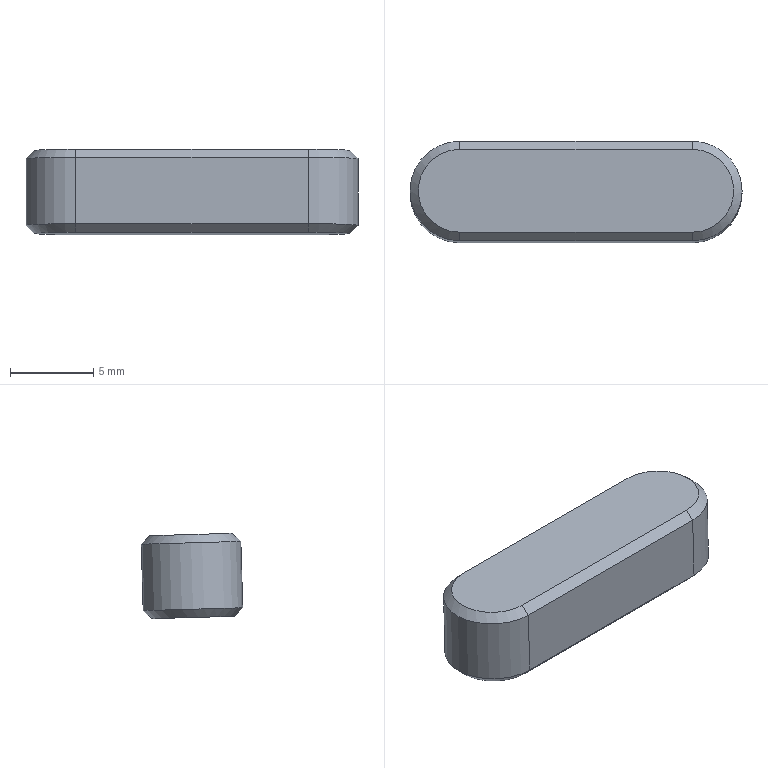Component | NX | KEY | 1 solid | 14 faces | box 20 x 6.11 x 5.14 mm | volume 550 mm3 | plane 8 | cone 4 | cylinder 2 | commonest cylinder face diameters 6 x2
STEP:
#1=CARTESIAN_POINT('',(0.,0.,0.));
#2=DIRECTION('',(0.,0.,1.));
#3=DIRECTION('',(1.,0.,0.));
#4=AXIS2_PLACEMENT_3D('',#1,#2,#3);
#5=CARTESIAN_POINT('',(-86.,-3.299,-0.9099));
#6=VERTEX_POINT('',#5);
#7=CARTESIAN_POINT('',(-86.,-3.185,3.088));
#8=VERTEX_POINT('',#7);
#9=CARTESIAN_POINT('',(-86.,-3.313,-1.41));
#10=DIRECTION('',(0.,0.0286,0.9996));
#11=VECTOR('',#10,1.);
#12=LINE('',#9,#11);
#13=CARTESIAN_POINT('',(-100.,-3.313,-1.41));
#14=DIRECTION('',(-0.,-0.9996,0.0286));
#15=DIRECTION('',(-1.,0.,-0.));
#16=AXIS2_PLACEMENT_3D('',#13,#14,#15);
#17=PLANE('',#16);
#18=CARTESIAN_POINT('',(-14.,0.));
#19=DIRECTION('',(0.,-1.));
#20=VECTOR('',#19,1.);
#21=LINE('',#18,#20);
#22=(GEOMETRIC_REPRESENTATION_CONTEXT(2)PARAMETRIC_REPRESENTATION_CONTEXT()REPRESENTATION_CONTEXT('',''));
#23=DEFINITIONAL_REPRESENTATION('',(#21),#22);
#24=PCURVE('',#17,#23);
#25=CARTESIAN_POINT('',(-86.,-0.3146,-1.495));
#26=DIRECTION('',(0.,0.0286,0.9996));
#27=DIRECTION('',(0.,0.9996,-0.0286));
#28=AXIS2_PLACEMENT_3D('',#25,#26,#27);
#29=CYLINDRICAL_SURFACE('',#28,3.);
#30=CARTESIAN_POINT('',(3.142,0.));
#31=DIRECTION('',(0.,1.));
#32=VECTOR('',#31,1.);
#33=LINE('',#30,#32);
#34=(GEOMETRIC_REPRESENTATION_CONTEXT(2)PARAMETRIC_REPRESENTATION_CONTEXT()REPRESENTATION_CONTEXT('',''));
#35=DEFINITIONAL_REPRESENTATION('',(#33),#34);
#36=PCURVE('',#29,#35);
#37=SURFACE_CURVE('',#12,(#24,#36),.PCURVE_S1.);
#38=EDGE_CURVE('',#6,#8,#37,.T.);
#39=ORIENTED_EDGE('',*,*,#38,.T.);
#40=CARTESIAN_POINT('',(-100.,-3.185,3.088));
#41=VERTEX_POINT('',#40);
#42=CARTESIAN_POINT('',(-100.,-3.185,3.088));
#43=DIRECTION('',(-1.,0.,-0.));
#44=VECTOR('',#43,1.);
#45=LINE('',#42,#44);
#46=CARTESIAN_POINT('',(0.,-4.5));
#47=DIRECTION('',(1.,0.));
#48=VECTOR('',#47,1.);
#49=LINE('',#46,#48);
#50=(GEOMETRIC_REPRESENTATION_CONTEXT(2)PARAMETRIC_REPRESENTATION_CONTEXT()REPRESENTATION_CONTEXT('',''));
#51=DEFINITIONAL_REPRESENTATION('',(#49),#50);
#52=PCURVE('',#17,#51);
#53=CARTESIAN_POINT('',(-86.,-2.671,3.574));
#54=DIRECTION('',(0.,0.6866,-0.727));
#55=DIRECTION('',(1.,-0.,0.));
#56=AXIS2_PLACEMENT_3D('',#53,#54,#55);
#57=PLANE('',#56);
#58=CARTESIAN_POINT('',(-14.,0.7071));
#59=DIRECTION('',(-1.,0.));
#60=VECTOR('',#59,1.);
#61=LINE('',#58,#60);
#62=(GEOMETRIC_REPRESENTATION_CONTEXT(2)PARAMETRIC_REPRESENTATION_CONTEXT()REPRESENTATION_CONTEXT('',''));
#63=DEFINITIONAL_REPRESENTATION('',(#61),#62);
#64=PCURVE('',#57,#63);
#65=SURFACE_CURVE('',#45,(#52,#64),.PCURVE_S1.);
#66=EDGE_CURVE('',#8,#41,#65,.T.);
#67=ORIENTED_EDGE('',*,*,#66,.T.);
#68=CARTESIAN_POINT('',(-100.,-3.299,-0.9099));
#69=VERTEX_POINT('',#68);
#70=CARTESIAN_POINT('',(-100.,-3.313,-1.41));
#71=DIRECTION('',(0.,0.0286,0.9996));
#72=VECTOR('',#71,1.);
#73=LINE('',#70,#72);
#74=CARTESIAN_POINT('',(0.,0.));
#75=DIRECTION('',(0.,-1.));
#76=VECTOR('',#75,1.);
#77=LINE('',#74,#76);
#78=(GEOMETRIC_REPRESENTATION_CONTEXT(2)PARAMETRIC_REPRESENTATION_CONTEXT()REPRESENTATION_CONTEXT('',''));
#79=DEFINITIONAL_REPRESENTATION('',(#77),#78);
#80=PCURVE('',#17,#79);
#81=CARTESIAN_POINT('',(-100.,-0.3146,-1.495));
#82=DIRECTION('',(0.,0.0286,0.9996));
#83=DIRECTION('',(0.,0.9996,-0.0286));
#84=AXIS2_PLACEMENT_3D('',#81,#82,#83);
#85=CYLINDRICAL_SURFACE('',#84,3.);
#86=CARTESIAN_POINT('',(3.142,0.));
#87=DIRECTION('',(0.,1.));
#88=VECTOR('',#87,1.);
#89=LINE('',#86,#88);
#90=(GEOMETRIC_REPRESENTATION_CONTEXT(2)PARAMETRIC_REPRESENTATION_CONTEXT()REPRESENTATION_CONTEXT('',''));
#91=DEFINITIONAL_REPRESENTATION('',(#89),#90);
#92=PCURVE('',#85,#91);
#93=SURFACE_CURVE('',#73,(#80,#92),.PCURVE_S1.);
#94=EDGE_CURVE('',#69,#41,#93,.T.);
#95=ORIENTED_EDGE('',*,*,#94,.F.);
#96=CARTESIAN_POINT('',(-86.,-3.299,-0.9099));
#97=DIRECTION('',(1.,-0.,0.));
#98=VECTOR('',#97,1.);
#99=LINE('',#96,#98);
#100=CARTESIAN_POINT('',(-14.,-0.5));
#101=DIRECTION('',(-1.,-0.));
#102=VECTOR('',#101,1.);
#103=LINE('',#100,#102);
#104=(GEOMETRIC_REPRESENTATION_CONTEXT(2)PARAMETRIC_REPRESENTATION_CONTEXT()REPRESENTATION_CONTEXT('',''));
#105=DEFINITIONAL_REPRESENTATION('',(#103),#104);
#106=PCURVE('',#17,#105);
#107=CARTESIAN_POINT('',(-100.,-3.299,-0.9099));
#108=DIRECTION('',(-0.,-0.727,-0.6866));
#109=DIRECTION('',(-1.,0.,-0.));
#110=AXIS2_PLACEMENT_3D('',#107,#108,#109);
#111=PLANE('',#110);
#112=CARTESIAN_POINT('',(-14.,0.));
#113=DIRECTION('',(-1.,0.));
#114=VECTOR('',#113,1.);
#115=LINE('',#112,#114);
#116=(GEOMETRIC_REPRESENTATION_CONTEXT(2)PARAMETRIC_REPRESENTATION_CONTEXT()REPRESENTATION_CONTEXT('',''));
#117=DEFINITIONAL_REPRESENTATION('',(#115),#116);
#118=PCURVE('',#111,#117);
#119=SURFACE_CURVE('',#99,(#106,#118),.PCURVE_S1.);
#120=EDGE_CURVE('',#69,#6,#119,.T.);
#121=ORIENTED_EDGE('',*,*,#120,.T.);
#122=EDGE_LOOP('',(#39,#67,#95,#121));
#123=FACE_BOUND('',#122,.T.);
#124=ADVANCED_FACE('',(#123),#17,.T.);
#125=CARTESIAN_POINT('',(-86.,2.698,-1.082));
#126=VERTEX_POINT('',#125);
#127=CARTESIAN_POINT('',(-86.,2.813,2.917));
#128=VERTEX_POINT('',#127);
#129=CARTESIAN_POINT('',(-86.,2.684,-1.581));
#130=DIRECTION('',(0.,0.0286,0.9996));
#131=VECTOR('',#130,1.);
#132=LINE('',#129,#131);
#133=CARTESIAN_POINT('',(6.283,0.));
#134=DIRECTION('',(0.,1.));
#135=VECTOR('',#134,1.);
#136=LINE('',#133,#135);
#137=(GEOMETRIC_REPRESENTATION_CONTEXT(2)PARAMETRIC_REPRESENTATION_CONTEXT()REPRESENTATION_CONTEXT('',''));
#138=DEFINITIONAL_REPRESENTATION('',(#136),#137);
#139=PCURVE('',#29,#138);
#140=CARTESIAN_POINT('',(-86.,2.684,-1.581));
#141=DIRECTION('',(-0.,0.9996,-0.0286));
#142=DIRECTION('',(1.,0.,-0.));
#143=AXIS2_PLACEMENT_3D('',#140,#141,#142);
#144=PLANE('',#143);
#145=CARTESIAN_POINT('',(0.,0.));
#146=DIRECTION('',(0.,-1.));
#147=VECTOR('',#146,1.);
#148=LINE('',#145,#147);
#149=(GEOMETRIC_REPRESENTATION_CONTEXT(2)PARAMETRIC_REPRESENTATION_CONTEXT()REPRESENTATION_CONTEXT('',''));
#150=DEFINITIONAL_REPRESENTATION('',(#148),#149);
#151=PCURVE('',#144,#150);
#152=SURFACE_CURVE('',#132,(#139,#151),.PCURVE_S1.);
#153=EDGE_CURVE('',#126,#128,#152,.T.);
#154=ORIENTED_EDGE('',*,*,#153,.T.);
#155=CARTESIAN_POINT('',(-86.,-0.1859,3.003));
#156=DIRECTION('',(0.,-0.0286,-0.9996));
#157=DIRECTION('',(0.,0.9996,-0.0286));
#158=AXIS2_PLACEMENT_3D('',#155,#156,#157);
#159=CIRCLE('',#158,3.);
#160=CARTESIAN_POINT('',(6.283,4.5));
#161=DIRECTION('',(-1.,0.));
#162=VECTOR('',#161,1.);
#163=LINE('',#160,#162);
#164=(GEOMETRIC_REPRESENTATION_CONTEXT(2)PARAMETRIC_REPRESENTATION_CONTEXT()REPRESENTATION_CONTEXT('',''));
#165=DEFINITIONAL_REPRESENTATION('',(#163),#164);
#166=PCURVE('',#29,#165);
#167=CARTESIAN_POINT('',(-86.,-0.1716,3.502));
#168=DIRECTION('',(0.,-0.0286,-0.9996));
#169=DIRECTION('',(0.,-0.9996,0.0286));
#170=AXIS2_PLACEMENT_3D('',#167,#168,#169);
#171=CONICAL_SURFACE('',#170,2.5,0.7854);
#172=CARTESIAN_POINT('',(3.142,0.5));
#173=DIRECTION('',(1.,0.));
#174=VECTOR('',#173,1.);
#175=LINE('',#172,#174);
#176=(GEOMETRIC_REPRESENTATION_CONTEXT(2)PARAMETRIC_REPRESENTATION_CONTEXT()REPRESENTATION_CONTEXT('',''));
#177=DEFINITIONAL_REPRESENTATION('',(#175),#176);
#178=PCURVE('',#171,#177);
#179=SURFACE_CURVE('',#159,(#166,#178),.PCURVE_S1.);
#180=EDGE_CURVE('',#128,#8,#179,.T.);
#181=ORIENTED_EDGE('',*,*,#180,.T.);
#182=ORIENTED_EDGE('',*,*,#38,.F.);
#183=CARTESIAN_POINT('',(-86.,-0.3003,-0.9957));
#184=DIRECTION('',(0.,0.0286,0.9996));
#185=DIRECTION('',(0.,0.9996,-0.0286));
#186=AXIS2_PLACEMENT_3D('',#183,#184,#185);
#187=CIRCLE('',#186,3.);
#188=CARTESIAN_POINT('',(0.,0.5));
#189=DIRECTION('',(1.,0.));
#190=VECTOR('',#189,1.);
#191=LINE('',#188,#190);
#192=(GEOMETRIC_REPRESENTATION_CONTEXT(2)PARAMETRIC_REPRESENTATION_CONTEXT()REPRESENTATION_CONTEXT('',''));
#193=DEFINITIONAL_REPRESENTATION('',(#191),#192);
#194=PCURVE('',#29,#193);
#195=CARTESIAN_POINT('',(-86.,-0.3003,-0.9957));
#196=DIRECTION('',(0.,0.0286,0.9996));
#197=DIRECTION('',(0.,0.9996,-0.0286));
#198=AXIS2_PLACEMENT_3D('',#195,#196,#197);
#199=CONICAL_SURFACE('',#198,3.,0.7854);
#200=CARTESIAN_POINT('',(0.,0.));
#201=DIRECTION('',(1.,0.));
#202=VECTOR('',#201,1.);
#203=LINE('',#200,#202);
#204=(GEOMETRIC_REPRESENTATION_CONTEXT(2)PARAMETRIC_REPRESENTATION_CONTEXT()REPRESENTATION_CONTEXT('',''));
#205=DEFINITIONAL_REPRESENTATION('',(#203),#204);
#206=PCURVE('',#199,#205);
#207=SURFACE_CURVE('',#187,(#194,#206),.PCURVE_S1.);
#208=EDGE_CURVE('',#6,#126,#207,.T.);
#209=ORIENTED_EDGE('',*,*,#208,.T.);
#210=EDGE_LOOP('',(#154,#181,#182,#209));
#211=FACE_BOUND('',#210,.T.);
#212=ADVANCED_FACE('',(#211),#29,.T.);
#213=CARTESIAN_POINT('',(-100.,2.698,-1.082));
#214=VERTEX_POINT('',#213);
#215=CARTESIAN_POINT('',(-100.,2.813,2.917));
#216=VERTEX_POINT('',#215);
#217=CARTESIAN_POINT('',(-100.,2.684,-1.581));
#218=DIRECTION('',(0.,0.0286,0.9996));
#219=VECTOR('',#218,1.);
#220=LINE('',#217,#219);
#221=CARTESIAN_POINT('',(-14.,0.));
#222=DIRECTION('',(0.,-1.));
#223=VECTOR('',#222,1.);
#224=LINE('',#221,#223);
#225=(GEOMETRIC_REPRESENTATION_CONTEXT(2)PARAMETRIC_REPRESENTATION_CONTEXT()REPRESENTATION_CONTEXT('',''));
#226=DEFINITIONAL_REPRESENTATION('',(#224),#225);
#227=PCURVE('',#144,#226);
#228=CARTESIAN_POINT('',(0.,0.));
#229=DIRECTION('',(0.,1.));
#230=VECTOR('',#229,1.);
#231=LINE('',#228,#230);
#232=(GEOMETRIC_REPRESENTATION_CONTEXT(2)PARAMETRIC_REPRESENTATION_CONTEXT()REPRESENTATION_CONTEXT('',''));
#233=DEFINITIONAL_REPRESENTATION('',(#231),#232);
#234=PCURVE('',#85,#233);
#235=SURFACE_CURVE('',#220,(#227,#234),.PCURVE_S1.);
#236=EDGE_CURVE('',#214,#216,#235,.T.);
#237=ORIENTED_EDGE('',*,*,#236,.T.);
#238=CARTESIAN_POINT('',(-86.,2.813,2.917));
#239=DIRECTION('',(1.,0.,-0.));
#240=VECTOR('',#239,1.);
#241=LINE('',#238,#240);
#242=CARTESIAN_POINT('',(0.,-4.5));
#243=DIRECTION('',(1.,0.));
#244=VECTOR('',#243,1.);
#245=LINE('',#242,#244);
#246=(GEOMETRIC_REPRESENTATION_CONTEXT(2)PARAMETRIC_REPRESENTATION_CONTEXT()REPRESENTATION_CONTEXT('',''));
#247=DEFINITIONAL_REPRESENTATION('',(#245),#246);
#248=PCURVE('',#144,#247);
#249=CARTESIAN_POINT('',(-86.,2.327,3.431));
#250=DIRECTION('',(0.,-0.727,-0.6866));
#251=DIRECTION('',(-1.,-0.,0.));
#252=AXIS2_PLACEMENT_3D('',#249,#250,#251);
#253=PLANE('',#252);
#254=CARTESIAN_POINT('',(0.,0.7071));
#255=DIRECTION('',(-1.,-0.));
#256=VECTOR('',#255,1.);
#257=LINE('',#254,#256);
#258=(GEOMETRIC_REPRESENTATION_CONTEXT(2)PARAMETRIC_REPRESENTATION_CONTEXT()REPRESENTATION_CONTEXT('',''));
#259=DEFINITIONAL_REPRESENTATION('',(#257),#258);
#260=PCURVE('',#253,#259);
#261=SURFACE_CURVE('',#241,(#248,#260),.PCURVE_S1.);
#262=EDGE_CURVE('',#216,#128,#261,.T.);
#263=ORIENTED_EDGE('',*,*,#262,.T.);
#264=ORIENTED_EDGE('',*,*,#153,.F.);
#265=CARTESIAN_POINT('',(-100.,2.698,-1.082));
#266=DIRECTION('',(-1.,-0.,0.));
#267=VECTOR('',#266,1.);
#268=LINE('',#265,#267);
#269=CARTESIAN_POINT('',(-14.,-0.5));
#270=DIRECTION('',(-1.,-0.));
#271=VECTOR('',#270,1.);
#272=LINE('',#269,#271);
#273=(GEOMETRIC_REPRESENTATION_CONTEXT(2)PARAMETRIC_REPRESENTATION_CONTEXT()REPRESENTATION_CONTEXT('',''));
#274=DEFINITIONAL_REPRESENTATION('',(#272),#273);
#275=PCURVE('',#144,#274);
#276=CARTESIAN_POINT('',(-86.,2.698,-1.082));
#277=DIRECTION('',(-0.,0.6866,-0.727));
#278=DIRECTION('',(1.,0.,-0.));
#279=AXIS2_PLACEMENT_3D('',#276,#277,#278);
#280=PLANE('',#279);
#281=CARTESIAN_POINT('',(-14.,-0.));
#282=DIRECTION('',(-1.,-0.));
#283=VECTOR('',#282,1.);
#284=LINE('',#281,#283);
#285=(GEOMETRIC_REPRESENTATION_CONTEXT(2)PARAMETRIC_REPRESENTATION_CONTEXT()REPRESENTATION_CONTEXT('',''));
#286=DEFINITIONAL_REPRESENTATION('',(#284),#285);
#287=PCURVE('',#280,#286);
#288=SURFACE_CURVE('',#268,(#275,#287),.PCURVE_S1.);
#289=EDGE_CURVE('',#126,#214,#288,.T.);
#290=ORIENTED_EDGE('',*,*,#289,.T.);
#291=EDGE_LOOP('',(#237,#263,#264,#290));
#292=FACE_BOUND('',#291,.T.);
#293=ADVANCED_FACE('',(#292),#144,.T.);
#294=ORIENTED_EDGE('',*,*,#94,.T.);
#295=CARTESIAN_POINT('',(-100.,-0.1859,3.003));
#296=DIRECTION('',(0.,-0.0286,-0.9996));
#297=DIRECTION('',(0.,0.9996,-0.0286));
#298=AXIS2_PLACEMENT_3D('',#295,#296,#297);
#299=CIRCLE('',#298,3.);
#300=CARTESIAN_POINT('',(6.283,4.5));
#301=DIRECTION('',(-1.,0.));
#302=VECTOR('',#301,1.);
#303=LINE('',#300,#302);
#304=(GEOMETRIC_REPRESENTATION_CONTEXT(2)PARAMETRIC_REPRESENTATION_CONTEXT()REPRESENTATION_CONTEXT('',''));
#305=DEFINITIONAL_REPRESENTATION('',(#303),#304);
#306=PCURVE('',#85,#305);
#307=CARTESIAN_POINT('',(-100.,-0.1716,3.502));
#308=DIRECTION('',(0.,-0.0286,-0.9996));
#309=DIRECTION('',(0.,-0.9996,0.0286));
#310=AXIS2_PLACEMENT_3D('',#307,#308,#309);
#311=CONICAL_SURFACE('',#310,2.5,0.7854);
#312=CARTESIAN_POINT('',(-3.142,0.5));
#313=DIRECTION('',(1.,0.));
#314=VECTOR('',#313,1.);
#315=LINE('',#312,#314);
#316=(GEOMETRIC_REPRESENTATION_CONTEXT(2)PARAMETRIC_REPRESENTATION_CONTEXT()REPRESENTATION_CONTEXT('',''));
#317=DEFINITIONAL_REPRESENTATION('',(#315),#316);
#318=PCURVE('',#311,#317);
#319=SURFACE_CURVE('',#299,(#306,#318),.PCURVE_S1.);
#320=EDGE_CURVE('',#41,#216,#319,.T.);
#321=ORIENTED_EDGE('',*,*,#320,.T.);
#322=ORIENTED_EDGE('',*,*,#236,.F.);
#323=CARTESIAN_POINT('',(-100.,-0.3003,-0.9957));
#324=DIRECTION('',(0.,0.0286,0.9996));
#325=DIRECTION('',(0.,0.9996,-0.0286));
#326=AXIS2_PLACEMENT_3D('',#323,#324,#325);
#327=CIRCLE('',#326,3.);
#328=CARTESIAN_POINT('',(0.,0.5));
#329=DIRECTION('',(1.,0.));
#330=VECTOR('',#329,1.);
#331=LINE('',#328,#330);
#332=(GEOMETRIC_REPRESENTATION_CONTEXT(2)PARAMETRIC_REPRESENTATION_CONTEXT()REPRESENTATION_CONTEXT('',''));
#333=DEFINITIONAL_REPRESENTATION('',(#331),#332);
#334=PCURVE('',#85,#333);
#335=CARTESIAN_POINT('',(-100.,-0.3003,-0.9957));
#336=DIRECTION('',(0.,0.0286,0.9996));
#337=DIRECTION('',(0.,0.9996,-0.0286));
#338=AXIS2_PLACEMENT_3D('',#335,#336,#337);
#339=CONICAL_SURFACE('',#338,3.,0.7854);
#340=CARTESIAN_POINT('',(0.,-0.));
#341=DIRECTION('',(1.,0.));
#342=VECTOR('',#341,1.);
#343=LINE('',#340,#342);
#344=(GEOMETRIC_REPRESENTATION_CONTEXT(2)PARAMETRIC_REPRESENTATION_CONTEXT()REPRESENTATION_CONTEXT('',''));
#345=DEFINITIONAL_REPRESENTATION('',(#343),#344);
#346=PCURVE('',#339,#345);
#347=SURFACE_CURVE('',#327,(#334,#346),.PCURVE_S1.);
#348=EDGE_CURVE('',#214,#69,#347,.T.);
#349=ORIENTED_EDGE('',*,*,#348,.T.);
#350=EDGE_LOOP('',(#294,#321,#322,#349));
#351=FACE_BOUND('',#350,.T.);
#352=ADVANCED_FACE('',(#351),#85,.T.);
#353=CARTESIAN_POINT('',(-86.,-2.814,-1.424));
#354=VERTEX_POINT('',#353);
#355=CARTESIAN_POINT('',(-100.,-2.814,-1.424));
#356=VERTEX_POINT('',#355);
#357=CARTESIAN_POINT('',(-100.,-2.814,-1.424));
#358=DIRECTION('',(-1.,0.,-0.));
#359=VECTOR('',#358,1.);
#360=LINE('',#357,#359);
#361=CARTESIAN_POINT('',(-86.,-0.3146,-1.495));
#362=DIRECTION('',(0.,0.0286,0.9996));
#363=DIRECTION('',(0.,0.9996,-0.0286));
#364=AXIS2_PLACEMENT_3D('',#361,#362,#363);
#365=PLANE('',#364);
#366=CARTESIAN_POINT('',(-2.5,14.));
#367=DIRECTION('',(0.,1.));
#368=VECTOR('',#367,1.);
#369=LINE('',#366,#368);
#370=(GEOMETRIC_REPRESENTATION_CONTEXT(2)PARAMETRIC_REPRESENTATION_CONTEXT()REPRESENTATION_CONTEXT('',''));
#371=DEFINITIONAL_REPRESENTATION('',(#369),#370);
#372=PCURVE('',#365,#371);
#373=CARTESIAN_POINT('',(0.,0.7071));
#374=DIRECTION('',(1.,-0.));
#375=VECTOR('',#374,1.);
#376=LINE('',#373,#375);
#377=(GEOMETRIC_REPRESENTATION_CONTEXT(2)PARAMETRIC_REPRESENTATION_CONTEXT()REPRESENTATION_CONTEXT('',''));
#378=DEFINITIONAL_REPRESENTATION('',(#376),#377);
#379=PCURVE('',#111,#378);
#380=SURFACE_CURVE('',#360,(#372,#379),.PCURVE_S1.);
#381=EDGE_CURVE('',#354,#356,#380,.T.);
#382=ORIENTED_EDGE('',*,*,#381,.T.);
#383=CARTESIAN_POINT('',(-100.,2.184,-1.567));
#384=VERTEX_POINT('',#383);
#385=CARTESIAN_POINT('',(-100.,-0.3146,-1.495));
#386=DIRECTION('',(0.,-0.0286,-0.9996));
#387=DIRECTION('',(0.,0.9996,-0.0286));
#388=AXIS2_PLACEMENT_3D('',#385,#386,#387);
#389=CIRCLE('',#388,2.5);
#390=CARTESIAN_POINT('',(2.5,14.));
#391=CARTESIAN_POINT('',(2.5,9.67));
#392=CARTESIAN_POINT('',(-1.25,11.835));
#393=CARTESIAN_POINT('',(-5.,14.));
#394=CARTESIAN_POINT('',(-1.25,16.165));
#395=CARTESIAN_POINT('',(2.5,18.33));
#396=CARTESIAN_POINT('',(2.5,14.));
#397=(BOUNDED_CURVE()B_SPLINE_CURVE(2,(#390,#391,#392,#393,#394,#395,#396),.UNSPECIFIED.,.T.,.F.)B_SPLINE_CURVE_WITH_KNOTS((1,2,2,2,2,1),(-2.094,0.,2.094,4.189,6.283,8.378),.UNSPECIFIED.)CURVE()GEOMETRIC_REPRESENTATION_ITEM()RATIONAL_B_SPLINE_CURVE((1.,0.5,1.,0.5,1.,0.5,1.))REPRESENTATION_ITEM(''));
#398=(GEOMETRIC_REPRESENTATION_CONTEXT(2)PARAMETRIC_REPRESENTATION_CONTEXT()REPRESENTATION_CONTEXT('',''));
#399=DEFINITIONAL_REPRESENTATION('',(#397),#398);
#400=PCURVE('',#365,#399);
#401=CARTESIAN_POINT('',(6.283,-0.5));
#402=DIRECTION('',(-1.,-0.));
#403=VECTOR('',#402,1.);
#404=LINE('',#401,#403);
#405=(GEOMETRIC_REPRESENTATION_CONTEXT(2)PARAMETRIC_REPRESENTATION_CONTEXT()REPRESENTATION_CONTEXT('',''));
#406=DEFINITIONAL_REPRESENTATION('',(#404),#405);
#407=PCURVE('',#339,#406);
#408=SURFACE_CURVE('',#389,(#400,#407),.PCURVE_S1.);
#409=EDGE_CURVE('',#356,#384,#408,.T.);
#410=ORIENTED_EDGE('',*,*,#409,.T.);
#411=CARTESIAN_POINT('',(-86.,2.184,-1.567));
#412=VERTEX_POINT('',#411);
#413=CARTESIAN_POINT('',(-86.,2.184,-1.567));
#414=DIRECTION('',(1.,0.,-0.));
#415=VECTOR('',#414,1.);
#416=LINE('',#413,#415);
#417=CARTESIAN_POINT('',(2.5,0.));
#418=DIRECTION('',(0.,-1.));
#419=VECTOR('',#418,1.);
#420=LINE('',#417,#419);
#421=(GEOMETRIC_REPRESENTATION_CONTEXT(2)PARAMETRIC_REPRESENTATION_CONTEXT()REPRESENTATION_CONTEXT('',''));
#422=DEFINITIONAL_REPRESENTATION('',(#420),#421);
#423=PCURVE('',#365,#422);
#424=CARTESIAN_POINT('',(0.,0.7071));
#425=DIRECTION('',(1.,0.));
#426=VECTOR('',#425,1.);
#427=LINE('',#424,#426);
#428=(GEOMETRIC_REPRESENTATION_CONTEXT(2)PARAMETRIC_REPRESENTATION_CONTEXT()REPRESENTATION_CONTEXT('',''));
#429=DEFINITIONAL_REPRESENTATION('',(#427),#428);
#430=PCURVE('',#280,#429);
#431=SURFACE_CURVE('',#416,(#423,#430),.PCURVE_S1.);
#432=EDGE_CURVE('',#384,#412,#431,.T.);
#433=ORIENTED_EDGE('',*,*,#432,.T.);
#434=CARTESIAN_POINT('',(-86.,-0.3146,-1.495));
#435=DIRECTION('',(0.,-0.0286,-0.9996));
#436=DIRECTION('',(0.,0.9996,-0.0286));
#437=AXIS2_PLACEMENT_3D('',#434,#435,#436);
#438=CIRCLE('',#437,2.5);
#439=CARTESIAN_POINT('',(2.5,0.));
#440=CARTESIAN_POINT('',(2.5,-4.33));
#441=CARTESIAN_POINT('',(-1.25,-2.165));
#442=CARTESIAN_POINT('',(-5.,-0.));
#443=CARTESIAN_POINT('',(-1.25,2.165));
#444=CARTESIAN_POINT('',(2.5,4.33));
#445=CARTESIAN_POINT('',(2.5,0.));
#446=(BOUNDED_CURVE()B_SPLINE_CURVE(2,(#439,#440,#441,#442,#443,#444,#445),.UNSPECIFIED.,.T.,.F.)B_SPLINE_CURVE_WITH_KNOTS((1,2,2,2,2,1),(-2.094,0.,2.094,4.189,6.283,8.378),.UNSPECIFIED.)CURVE()GEOMETRIC_REPRESENTATION_ITEM()RATIONAL_B_SPLINE_CURVE((1.,0.5,1.,0.5,1.,0.5,1.))REPRESENTATION_ITEM(''));
#447=(GEOMETRIC_REPRESENTATION_CONTEXT(2)PARAMETRIC_REPRESENTATION_CONTEXT()REPRESENTATION_CONTEXT('',''));
#448=DEFINITIONAL_REPRESENTATION('',(#446),#447);
#449=PCURVE('',#365,#448);
#450=CARTESIAN_POINT('',(6.283,-0.5));
#451=DIRECTION('',(-1.,-0.));
#452=VECTOR('',#451,1.);
#453=LINE('',#450,#452);
#454=(GEOMETRIC_REPRESENTATION_CONTEXT(2)PARAMETRIC_REPRESENTATION_CONTEXT()REPRESENTATION_CONTEXT('',''));
#455=DEFINITIONAL_REPRESENTATION('',(#453),#454);
#456=PCURVE('',#199,#455);
#457=SURFACE_CURVE('',#438,(#449,#456),.PCURVE_S1.);
#458=EDGE_CURVE('',#412,#354,#457,.T.);
#459=ORIENTED_EDGE('',*,*,#458,.T.);
#460=EDGE_LOOP('',(#382,#410,#433,#459));
#461=FACE_BOUND('',#460,.T.);
#462=ADVANCED_FACE('',(#461),#365,.F.);
#463=CARTESIAN_POINT('',(-86.,2.327,3.431));
#464=VERTEX_POINT('',#463);
#465=CARTESIAN_POINT('',(-100.,2.327,3.431));
#466=VERTEX_POINT('',#465);
#467=CARTESIAN_POINT('',(-86.,2.327,3.431));
#468=DIRECTION('',(-1.,-0.,0.));
#469=VECTOR('',#468,1.);
#470=LINE('',#467,#469);
#471=CARTESIAN_POINT('',(-86.,-0.1716,3.502));
#472=DIRECTION('',(0.,0.0286,0.9996));
#473=DIRECTION('',(0.,0.9996,-0.0286));
#474=AXIS2_PLACEMENT_3D('',#471,#472,#473);
#475=PLANE('',#474);
#476=CARTESIAN_POINT('',(2.5,0.));
#477=DIRECTION('',(-0.,1.));
#478=VECTOR('',#477,1.);
#479=LINE('',#476,#478);
#480=(GEOMETRIC_REPRESENTATION_CONTEXT(2)PARAMETRIC_REPRESENTATION_CONTEXT()REPRESENTATION_CONTEXT('',''));
#481=DEFINITIONAL_REPRESENTATION('',(#479),#480);
#482=PCURVE('',#475,#481);
#483=CARTESIAN_POINT('',(0.,0.));
#484=DIRECTION('',(1.,0.));
#485=VECTOR('',#484,1.);
#486=LINE('',#483,#485);
#487=(GEOMETRIC_REPRESENTATION_CONTEXT(2)PARAMETRIC_REPRESENTATION_CONTEXT()REPRESENTATION_CONTEXT('',''));
#488=DEFINITIONAL_REPRESENTATION('',(#486),#487);
#489=PCURVE('',#253,#488);
#490=SURFACE_CURVE('',#470,(#482,#489),.PCURVE_S1.);
#491=EDGE_CURVE('',#464,#466,#490,.T.);
#492=ORIENTED_EDGE('',*,*,#491,.T.);
#493=CARTESIAN_POINT('',(-100.,-2.671,3.574));
#494=VERTEX_POINT('',#493);
#495=CARTESIAN_POINT('',(-100.,-0.1716,3.502));
#496=DIRECTION('',(0.,0.0286,0.9996));
#497=DIRECTION('',(0.,0.9996,-0.0286));
#498=AXIS2_PLACEMENT_3D('',#495,#496,#497);
#499=CIRCLE('',#498,2.5);
#500=CARTESIAN_POINT('',(0.,14.));
#501=DIRECTION('',(1.,0.));
#502=AXIS2_PLACEMENT_2D('',#500,#501);
#503=CIRCLE('',#502,2.5);
#504=(GEOMETRIC_REPRESENTATION_CONTEXT(2)PARAMETRIC_REPRESENTATION_CONTEXT()REPRESENTATION_CONTEXT('',''));
#505=DEFINITIONAL_REPRESENTATION('',(#503),#504);
#506=PCURVE('',#475,#505);
#507=CARTESIAN_POINT('',(3.142,0.));
#508=DIRECTION('',(-1.,0.));
#509=VECTOR('',#508,1.);
#510=LINE('',#507,#509);
#511=(GEOMETRIC_REPRESENTATION_CONTEXT(2)PARAMETRIC_REPRESENTATION_CONTEXT()REPRESENTATION_CONTEXT('',''));
#512=DEFINITIONAL_REPRESENTATION('',(#510),#511);
#513=PCURVE('',#311,#512);
#514=SURFACE_CURVE('',#499,(#506,#513),.PCURVE_S1.);
#515=EDGE_CURVE('',#466,#494,#514,.T.);
#516=ORIENTED_EDGE('',*,*,#515,.T.);
#517=CARTESIAN_POINT('',(-86.,-2.671,3.574));
#518=VERTEX_POINT('',#517);
#519=CARTESIAN_POINT('',(-86.,-2.671,3.574));
#520=DIRECTION('',(1.,-0.,0.));
#521=VECTOR('',#520,1.);
#522=LINE('',#519,#521);
#523=CARTESIAN_POINT('',(-2.5,0.));
#524=DIRECTION('',(-0.,-1.));
#525=VECTOR('',#524,1.);
#526=LINE('',#523,#525);
#527=(GEOMETRIC_REPRESENTATION_CONTEXT(2)PARAMETRIC_REPRESENTATION_CONTEXT()REPRESENTATION_CONTEXT('',''));
#528=DEFINITIONAL_REPRESENTATION('',(#526),#527);
#529=PCURVE('',#475,#528);
#530=CARTESIAN_POINT('',(0.,0.));
#531=DIRECTION('',(1.,-0.));
#532=VECTOR('',#531,1.);
#533=LINE('',#530,#532);
#534=(GEOMETRIC_REPRESENTATION_CONTEXT(2)PARAMETRIC_REPRESENTATION_CONTEXT()REPRESENTATION_CONTEXT('',''));
#535=DEFINITIONAL_REPRESENTATION('',(#533),#534);
#536=PCURVE('',#57,#535);
#537=SURFACE_CURVE('',#522,(#529,#536),.PCURVE_S1.);
#538=EDGE_CURVE('',#494,#518,#537,.T.);
#539=ORIENTED_EDGE('',*,*,#538,.T.);
#540=CARTESIAN_POINT('',(-86.,-0.1716,3.502));
#541=DIRECTION('',(0.,0.0286,0.9996));
#542=DIRECTION('',(0.,0.9996,-0.0286));
#543=AXIS2_PLACEMENT_3D('',#540,#541,#542);
#544=CIRCLE('',#543,2.5);
#545=CARTESIAN_POINT('',(0.,0.));
#546=DIRECTION('',(1.,0.));
#547=AXIS2_PLACEMENT_2D('',#545,#546);
#548=CIRCLE('',#547,2.5);
#549=(GEOMETRIC_REPRESENTATION_CONTEXT(2)PARAMETRIC_REPRESENTATION_CONTEXT()REPRESENTATION_CONTEXT('',''));
#550=DEFINITIONAL_REPRESENTATION('',(#548),#549);
#551=PCURVE('',#475,#550);
#552=CARTESIAN_POINT('',(9.425,0.));
#553=DIRECTION('',(-1.,0.));
#554=VECTOR('',#553,1.);
#555=LINE('',#552,#554);
#556=(GEOMETRIC_REPRESENTATION_CONTEXT(2)PARAMETRIC_REPRESENTATION_CONTEXT()REPRESENTATION_CONTEXT('',''));
#557=DEFINITIONAL_REPRESENTATION('',(#555),#556);
#558=PCURVE('',#171,#557);
#559=SURFACE_CURVE('',#544,(#551,#558),.PCURVE_S1.);
#560=EDGE_CURVE('',#518,#464,#559,.T.);
#561=ORIENTED_EDGE('',*,*,#560,.T.);
#562=EDGE_LOOP('',(#492,#516,#539,#561));
#563=FACE_BOUND('',#562,.T.);
#564=ADVANCED_FACE('',(#563),#475,.T.);
#565=CARTESIAN_POINT('',(-86.,-3.185,3.088));
#566=DIRECTION('',(0.,0.727,0.6866));
#567=VECTOR('',#566,1.);
#568=LINE('',#565,#567);
#569=CARTESIAN_POINT('',(6.283,0.5));
#570=DIRECTION('',(0.,-1.));
#571=VECTOR('',#570,1.);
#572=LINE('',#569,#571);
#573=(GEOMETRIC_REPRESENTATION_CONTEXT(2)PARAMETRIC_REPRESENTATION_CONTEXT()REPRESENTATION_CONTEXT('',''));
#574=DEFINITIONAL_REPRESENTATION('',(#572),#573);
#575=PCURVE('',#171,#574);
#576=CARTESIAN_POINT('',(-0.,0.7071));
#577=DIRECTION('',(0.,-1.));
#578=VECTOR('',#577,1.);
#579=LINE('',#576,#578);
#580=(GEOMETRIC_REPRESENTATION_CONTEXT(2)PARAMETRIC_REPRESENTATION_CONTEXT()REPRESENTATION_CONTEXT('',''));
#581=DEFINITIONAL_REPRESENTATION('',(#579),#580);
#582=PCURVE('',#57,#581);
#583=SURFACE_CURVE('',#568,(#575,#582),.PCURVE_S1.);
#584=EDGE_CURVE('',#8,#518,#583,.T.);
#585=ORIENTED_EDGE('',*,*,#584,.F.);
#586=ORIENTED_EDGE('',*,*,#180,.F.);
#587=CARTESIAN_POINT('',(-86.,2.327,3.431));
#588=DIRECTION('',(-0.,0.6866,-0.727));
#589=VECTOR('',#588,1.);
#590=LINE('',#587,#589);
#591=CARTESIAN_POINT('',(3.142,-0.));
#592=DIRECTION('',(0.,1.));
#593=VECTOR('',#592,1.);
#594=LINE('',#591,#593);
#595=(GEOMETRIC_REPRESENTATION_CONTEXT(2)PARAMETRIC_REPRESENTATION_CONTEXT()REPRESENTATION_CONTEXT('',''));
#596=DEFINITIONAL_REPRESENTATION('',(#594),#595);
#597=PCURVE('',#171,#596);
#598=CARTESIAN_POINT('',(0.,0.));
#599=DIRECTION('',(-0.,1.));
#600=VECTOR('',#599,1.);
#601=LINE('',#598,#600);
#602=(GEOMETRIC_REPRESENTATION_CONTEXT(2)PARAMETRIC_REPRESENTATION_CONTEXT()REPRESENTATION_CONTEXT('',''));
#603=DEFINITIONAL_REPRESENTATION('',(#601),#602);
#604=PCURVE('',#253,#603);
#605=SURFACE_CURVE('',#590,(#597,#604),.PCURVE_S1.);
#606=EDGE_CURVE('',#464,#128,#605,.T.);
#607=ORIENTED_EDGE('',*,*,#606,.F.);
#608=ORIENTED_EDGE('',*,*,#560,.F.);
#609=EDGE_LOOP('',(#585,#586,#607,#608));
#610=FACE_BOUND('',#609,.T.);
#611=ADVANCED_FACE('',(#610),#171,.T.);
#612=ORIENTED_EDGE('',*,*,#606,.T.);
#613=ORIENTED_EDGE('',*,*,#262,.F.);
#614=CARTESIAN_POINT('',(-100.,2.327,3.431));
#615=DIRECTION('',(0.,0.6866,-0.727));
#616=VECTOR('',#615,1.);
#617=LINE('',#614,#616);
#618=CARTESIAN_POINT('',(14.,0.));
#619=DIRECTION('',(-0.,1.));
#620=VECTOR('',#619,1.);
#621=LINE('',#618,#620);
#622=(GEOMETRIC_REPRESENTATION_CONTEXT(2)PARAMETRIC_REPRESENTATION_CONTEXT()REPRESENTATION_CONTEXT('',''));
#623=DEFINITIONAL_REPRESENTATION('',(#621),#622);
#624=PCURVE('',#253,#623);
#625=CARTESIAN_POINT('',(3.142,-0.));
#626=DIRECTION('',(0.,1.));
#627=VECTOR('',#626,1.);
#628=LINE('',#625,#627);
#629=(GEOMETRIC_REPRESENTATION_CONTEXT(2)PARAMETRIC_REPRESENTATION_CONTEXT()REPRESENTATION_CONTEXT('',''));
#630=DEFINITIONAL_REPRESENTATION('',(#628),#629);
#631=PCURVE('',#311,#630);
#632=SURFACE_CURVE('',#617,(#624,#631),.PCURVE_S1.);
#633=EDGE_CURVE('',#466,#216,#632,.T.);
#634=ORIENTED_EDGE('',*,*,#633,.F.);
#635=ORIENTED_EDGE('',*,*,#491,.F.);
#636=EDGE_LOOP('',(#612,#613,#634,#635));
#637=FACE_BOUND('',#636,.T.);
#638=ADVANCED_FACE('',(#637),#253,.F.);
#639=ORIENTED_EDGE('',*,*,#584,.T.);
#640=ORIENTED_EDGE('',*,*,#538,.F.);
#641=CARTESIAN_POINT('',(-100.,-3.185,3.088));
#642=DIRECTION('',(0.,0.727,0.6866));
#643=VECTOR('',#642,1.);
#644=LINE('',#641,#643);
#645=CARTESIAN_POINT('',(-14.,0.7071));
#646=DIRECTION('',(-0.,-1.));
#647=VECTOR('',#646,1.);
#648=LINE('',#645,#647);
#649=(GEOMETRIC_REPRESENTATION_CONTEXT(2)PARAMETRIC_REPRESENTATION_CONTEXT()REPRESENTATION_CONTEXT('',''));
#650=DEFINITIONAL_REPRESENTATION('',(#648),#649);
#651=PCURVE('',#57,#650);
#652=CARTESIAN_POINT('',(0.,0.5));
#653=DIRECTION('',(0.,-1.));
#654=VECTOR('',#653,1.);
#655=LINE('',#652,#654);
#656=(GEOMETRIC_REPRESENTATION_CONTEXT(2)PARAMETRIC_REPRESENTATION_CONTEXT()REPRESENTATION_CONTEXT('',''));
#657=DEFINITIONAL_REPRESENTATION('',(#655),#656);
#658=PCURVE('',#311,#657);
#659=SURFACE_CURVE('',#644,(#651,#658),.PCURVE_S1.);
#660=EDGE_CURVE('',#41,#494,#659,.T.);
#661=ORIENTED_EDGE('',*,*,#660,.F.);
#662=ORIENTED_EDGE('',*,*,#66,.F.);
#663=EDGE_LOOP('',(#639,#640,#661,#662));
#664=FACE_BOUND('',#663,.T.);
#665=ADVANCED_FACE('',(#664),#57,.F.);
#666=ORIENTED_EDGE('',*,*,#633,.T.);
#667=ORIENTED_EDGE('',*,*,#320,.F.);
#668=ORIENTED_EDGE('',*,*,#660,.T.);
#669=ORIENTED_EDGE('',*,*,#515,.F.);
#670=EDGE_LOOP('',(#666,#667,#668,#669));
#671=FACE_BOUND('',#670,.T.);
#672=ADVANCED_FACE('',(#671),#311,.T.);
#673=CARTESIAN_POINT('',(-86.,-2.814,-1.424));
#674=DIRECTION('',(-0.,-0.6866,0.727));
#675=VECTOR('',#674,1.);
#676=LINE('',#673,#675);
#677=CARTESIAN_POINT('',(3.142,-0.5));
#678=DIRECTION('',(-0.,1.));
#679=VECTOR('',#678,1.);
#680=LINE('',#677,#679);
#681=(GEOMETRIC_REPRESENTATION_CONTEXT(2)PARAMETRIC_REPRESENTATION_CONTEXT()REPRESENTATION_CONTEXT('',''));
#682=DEFINITIONAL_REPRESENTATION('',(#680),#681);
#683=PCURVE('',#199,#682);
#684=CARTESIAN_POINT('',(-14.,0.7071));
#685=DIRECTION('',(0.,-1.));
#686=VECTOR('',#685,1.);
#687=LINE('',#684,#686);
#688=(GEOMETRIC_REPRESENTATION_CONTEXT(2)PARAMETRIC_REPRESENTATION_CONTEXT()REPRESENTATION_CONTEXT('',''));
#689=DEFINITIONAL_REPRESENTATION('',(#687),#688);
#690=PCURVE('',#111,#689);
#691=SURFACE_CURVE('',#676,(#683,#690),.PCURVE_S1.);
#692=EDGE_CURVE('',#354,#6,#691,.T.);
#693=ORIENTED_EDGE('',*,*,#692,.F.);
#694=ORIENTED_EDGE('',*,*,#458,.F.);
#695=CARTESIAN_POINT('',(-86.,2.698,-1.082));
#696=DIRECTION('',(0.,-0.727,-0.6866));
#697=VECTOR('',#696,1.);
#698=LINE('',#695,#697);
#699=CARTESIAN_POINT('',(6.283,0.));
#700=DIRECTION('',(0.,-1.));
#701=VECTOR('',#700,1.);
#702=LINE('',#699,#701);
#703=(GEOMETRIC_REPRESENTATION_CONTEXT(2)PARAMETRIC_REPRESENTATION_CONTEXT()REPRESENTATION_CONTEXT('',''));
#704=DEFINITIONAL_REPRESENTATION('',(#702),#703);
#705=PCURVE('',#199,#704);
#706=CARTESIAN_POINT('',(0.,0.));
#707=DIRECTION('',(-0.,1.));
#708=VECTOR('',#707,1.);
#709=LINE('',#706,#708);
#710=(GEOMETRIC_REPRESENTATION_CONTEXT(2)PARAMETRIC_REPRESENTATION_CONTEXT()REPRESENTATION_CONTEXT('',''));
#711=DEFINITIONAL_REPRESENTATION('',(#709),#710);
#712=PCURVE('',#280,#711);
#713=SURFACE_CURVE('',#698,(#705,#712),.PCURVE_S1.);
#714=EDGE_CURVE('',#126,#412,#713,.T.);
#715=ORIENTED_EDGE('',*,*,#714,.F.);
#716=ORIENTED_EDGE('',*,*,#208,.F.);
#717=EDGE_LOOP('',(#693,#694,#715,#716));
#718=FACE_BOUND('',#717,.T.);
#719=ADVANCED_FACE('',(#718),#199,.T.);
#720=ORIENTED_EDGE('',*,*,#714,.T.);
#721=ORIENTED_EDGE('',*,*,#432,.F.);
#722=CARTESIAN_POINT('',(-100.,2.698,-1.082));
#723=DIRECTION('',(0.,-0.727,-0.6866));
#724=VECTOR('',#723,1.);
#725=LINE('',#722,#724);
#726=CARTESIAN_POINT('',(-14.,-0.));
#727=DIRECTION('',(-0.,1.));
#728=VECTOR('',#727,1.);
#729=LINE('',#726,#728);
#730=(GEOMETRIC_REPRESENTATION_CONTEXT(2)PARAMETRIC_REPRESENTATION_CONTEXT()REPRESENTATION_CONTEXT('',''));
#731=DEFINITIONAL_REPRESENTATION('',(#729),#730);
#732=PCURVE('',#280,#731);
#733=CARTESIAN_POINT('',(0.,-0.));
#734=DIRECTION('',(0.,-1.));
#735=VECTOR('',#734,1.);
#736=LINE('',#733,#735);
#737=(GEOMETRIC_REPRESENTATION_CONTEXT(2)PARAMETRIC_REPRESENTATION_CONTEXT()REPRESENTATION_CONTEXT('',''));
#738=DEFINITIONAL_REPRESENTATION('',(#736),#737);
#739=PCURVE('',#339,#738);
#740=SURFACE_CURVE('',#725,(#732,#739),.PCURVE_S1.);
#741=EDGE_CURVE('',#214,#384,#740,.T.);
#742=ORIENTED_EDGE('',*,*,#741,.F.);
#743=ORIENTED_EDGE('',*,*,#289,.F.);
#744=EDGE_LOOP('',(#720,#721,#742,#743));
#745=FACE_BOUND('',#744,.T.);
#746=ADVANCED_FACE('',(#745),#280,.T.);
#747=ORIENTED_EDGE('',*,*,#692,.T.);
#748=ORIENTED_EDGE('',*,*,#120,.F.);
#749=CARTESIAN_POINT('',(-100.,-2.814,-1.424));
#750=DIRECTION('',(0.,-0.6866,0.727));
#751=VECTOR('',#750,1.);
#752=LINE('',#749,#751);
#753=CARTESIAN_POINT('',(0.,0.7071));
#754=DIRECTION('',(-0.,-1.));
#755=VECTOR('',#754,1.);
#756=LINE('',#753,#755);
#757=(GEOMETRIC_REPRESENTATION_CONTEXT(2)PARAMETRIC_REPRESENTATION_CONTEXT()REPRESENTATION_CONTEXT('',''));
#758=DEFINITIONAL_REPRESENTATION('',(#756),#757);
#759=PCURVE('',#111,#758);
#760=CARTESIAN_POINT('',(3.142,-0.5));
#761=DIRECTION('',(0.,1.));
#762=VECTOR('',#761,1.);
#763=LINE('',#760,#762);
#764=(GEOMETRIC_REPRESENTATION_CONTEXT(2)PARAMETRIC_REPRESENTATION_CONTEXT()REPRESENTATION_CONTEXT('',''));
#765=DEFINITIONAL_REPRESENTATION('',(#763),#764);
#766=PCURVE('',#339,#765);
#767=SURFACE_CURVE('',#752,(#759,#766),.PCURVE_S1.);
#768=EDGE_CURVE('',#356,#69,#767,.T.);
#769=ORIENTED_EDGE('',*,*,#768,.F.);
#770=ORIENTED_EDGE('',*,*,#381,.F.);
#771=EDGE_LOOP('',(#747,#748,#769,#770));
#772=FACE_BOUND('',#771,.T.);
#773=ADVANCED_FACE('',(#772),#111,.T.);
#774=ORIENTED_EDGE('',*,*,#741,.T.);
#775=ORIENTED_EDGE('',*,*,#409,.F.);
#776=ORIENTED_EDGE('',*,*,#768,.T.);
#777=ORIENTED_EDGE('',*,*,#348,.F.);
#778=EDGE_LOOP('',(#774,#775,#776,#777));
#779=FACE_BOUND('',#778,.T.);
#780=ADVANCED_FACE('',(#779),#339,.T.);
#781=CLOSED_SHELL('',(#124,#212,#293,#352,#462,#564,#611,#638,#665,#672,#719,#746,#773,#780));
#782=MANIFOLD_SOLID_BREP('',#781);
#783=(LENGTH_UNIT()NAMED_UNIT(*)SI_UNIT(.MILLI.,.METRE.));
#784=UNCERTAINTY_MEASURE_WITH_UNIT(LENGTH_MEASURE(0.0000001),#783,'','');
#785=(NAMED_UNIT(*)PLANE_ANGLE_UNIT()SI_UNIT($,.RADIAN.));
#786=(NAMED_UNIT(*)SI_UNIT($,.STERADIAN.)SOLID_ANGLE_UNIT());
#787=(GEOMETRIC_REPRESENTATION_CONTEXT(3)GLOBAL_UNCERTAINTY_ASSIGNED_CONTEXT((#784))GLOBAL_UNIT_ASSIGNED_CONTEXT((#783,#785,#786))REPRESENTATION_CONTEXT('',''));
#788=ADVANCED_BREP_SHAPE_REPRESENTATION('',(#4,#782),#787);